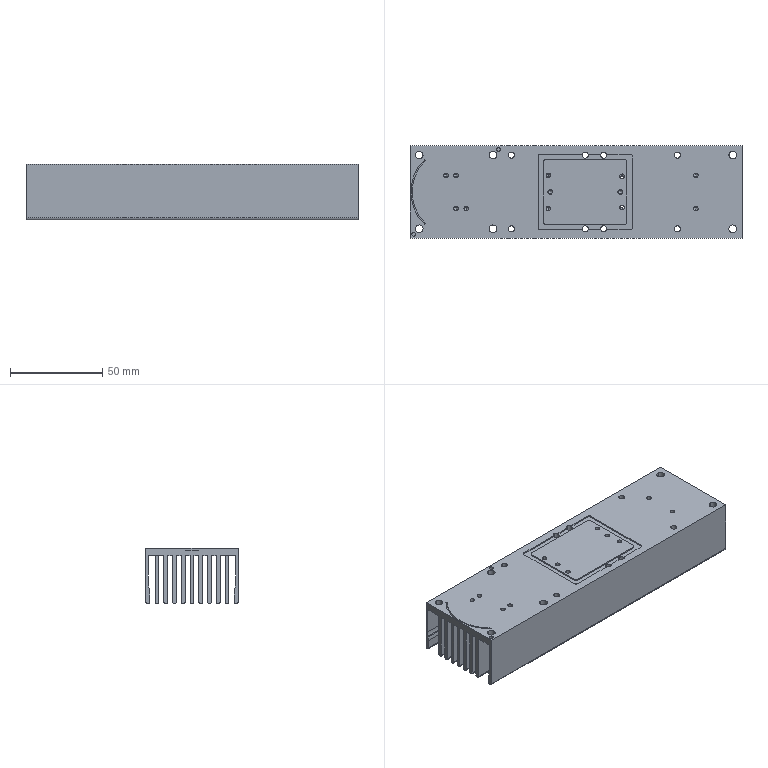CAM job | Mastercam | mm | 14 operations | part box 180 x 50 x 30
1. Drill/Counterbore | 4 - 6 倒角刀
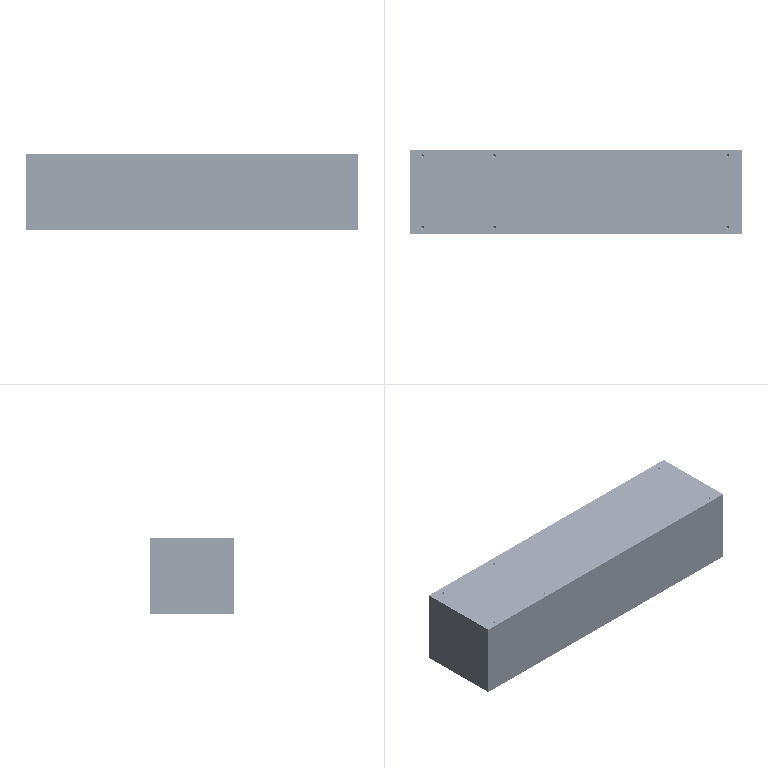2. Drill/Counterbore | 4 - 6 倒角刀
3. Drill/Counterbore | 4 - 6 倒角刀
4. Peck Drill | 19 - 4.2 钻头
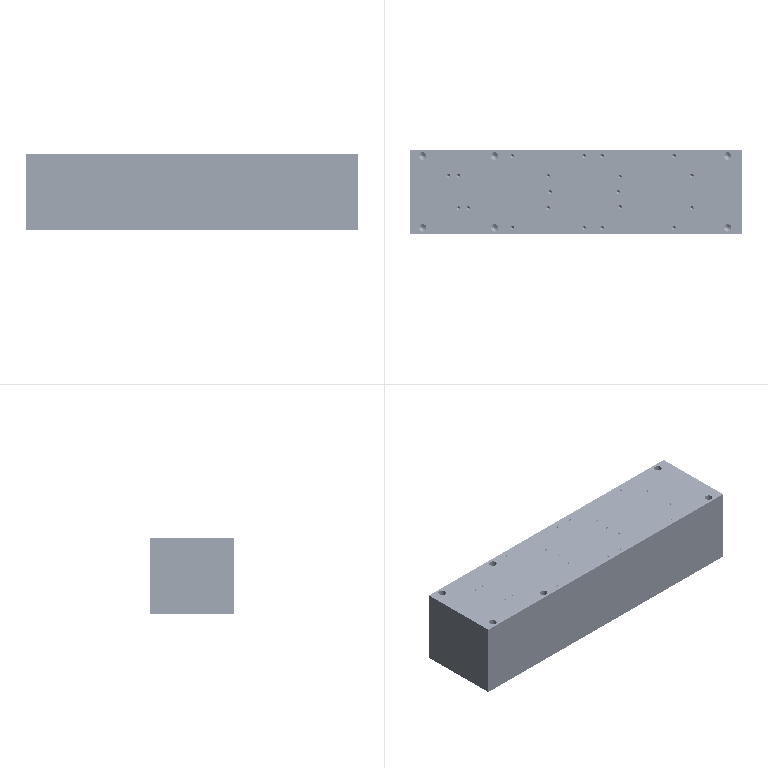5. Peck Drill | 12 - 3.3 钻头
6. Peck Drill | 5 - 2.5 钻头
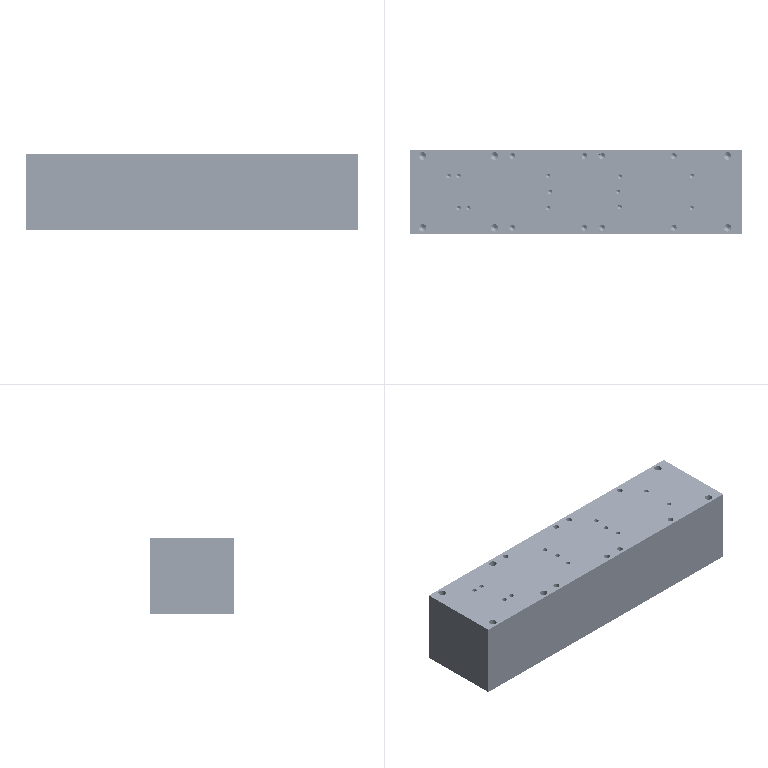7. Contour (Ramp) | 28 - 1.5 平铣刀
8. Contour (2D) | 28 - 1.5 平铣刀
9. 2D High Speed (2D Area Mill) | 14 - 2 平铣刀
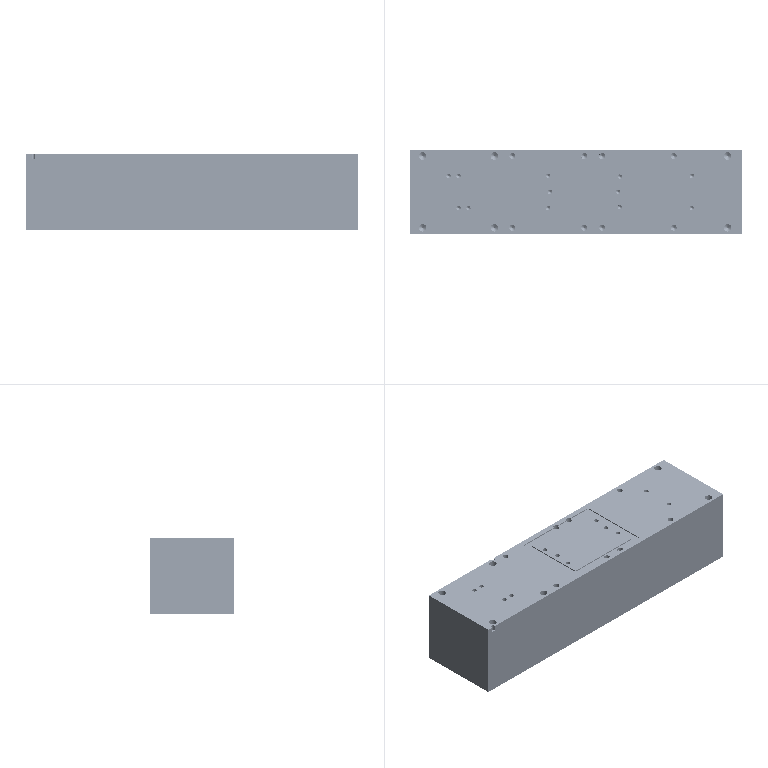10. Contour (2D) | 15 - 2J
11. Contour (Ramp) | 29 - 0.6 平铣刀
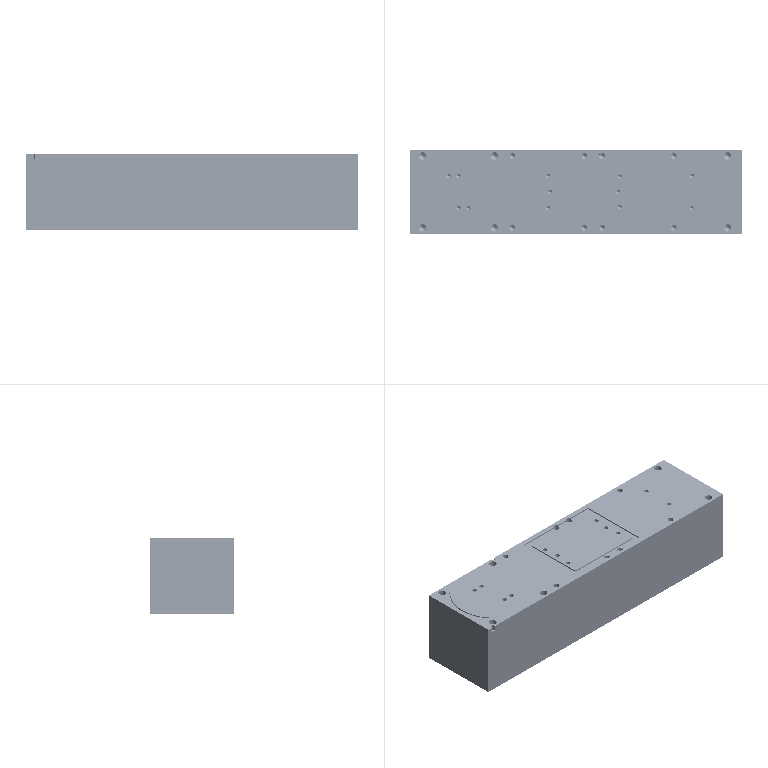12. Model Chamfer | 4 - 6 倒角刀
13. 2D High Speed (2D Area Mill) | 7 - 4 平铣刀
14. Contour (2D) | 8 - 4J